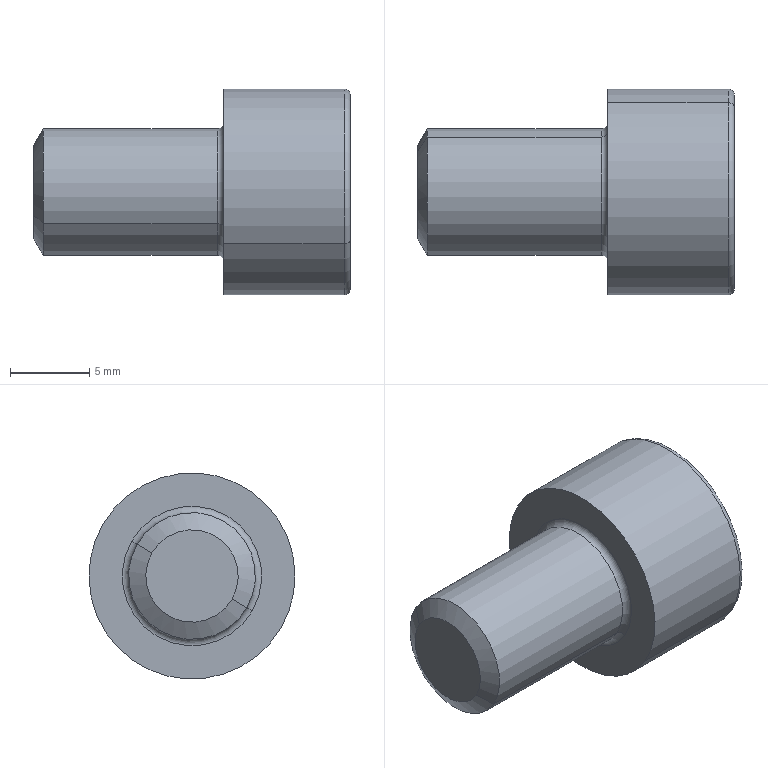Component | NX | HEX_SOCKET_CAP_SCREW_M8X12_10 | 1 solid | 20 faces | volume 1535 mm3 | plane 10 | torus 4 | cylinder 4 | cone 2 | commonest cylinder face diameters 13 x2 8 x2